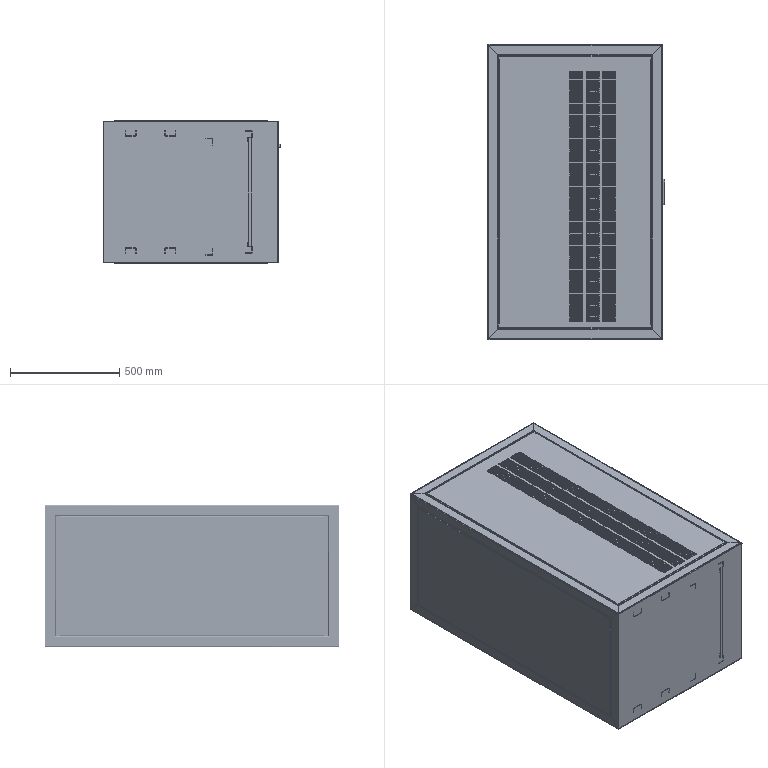Assembly | SolidWorks | mm | 39 component files | 39 solids | 4179 faces | box 814 x 1350 x 654 mm | volume 14968094 mm3 | plane 2169 | cylinder 1888 | spline 120 | torus 2 | commonest cylinder face diameters 5 x1380 8 x288 4 x90 6.4 x48 10 x28 6 x28 6.5 x12 7 x6
Bill of materials:
AuxiliaryPanel1 | 1 |  | Long thin-walled C-channel (lipped channel) profile with a flat web, two short flanges with rounded bends, and short inward-turned return lips; constant cross-section along its length.
AuxiliaryPanel2 | 1 |  | Long thin-walled lipped C-channel profile, similar to a sheet-formed channel, with flat web, rounded bends, short flanges and inward return lips; a single small round hole is visible near one end of a flange.
Beam1.1 | 1 |  | Straight angle profile (L-section) with two legs of roughly equal length joined by a rounded inside/outside bend; constant cross-section with plain square-cut ends.
Beam1.2 | 1 |  | Straight angle profile (L-section) with roughly equal legs and a radiused bend, shown with the corner facing the viewer; constant cross-section and plain ends.
Beam1.3 | 1 |  | Straight angle profile (L-section) with roughly equal legs and a radiused bend; plain ends, uniform cross-section.
Beam1.4 | 1 |  | Straight angle profile (L-section) with roughly equal legs and a radiused bend, corner facing the viewer; plain ends.
Beam1.5 | 1 |  | Straight angle profile (L-section) with roughly equal legs and a radiused bend, corner facing the viewer; plain ends.
Beam1.6 | 1 |  | Straight angle profile (L-section) with roughly equal legs and a radiused bend; plain ends, uniform cross-section.
BottomSupport | 3 |  | Long, thin rectangular flat bar or strip with small rounded or chamfered edges along its long sides; no holes or cut-outs visible.
FrontAndRearPlate1 | 1 |  | Thin sheet-formed Z-shaped (joggled) profile: two parallel offset flanges connected by a short web with rounded bends; the ends are cut at an angle so the outline narrows at the top and bottom.
FrontAndRearPlate2 | 1 |  | Thin sheet-formed Z-shaped (joggled) profile with angled cut ends, similar to unnamed part but mirrored in section; one small round hole near one end of a flange.
FrontAndRearPlate3 | 1 |  | Thin sheet-formed Z-shaped (joggled) profile with angled cut ends and one small round hole near one end of a flange; appears to be a mirrored or reoriented version of the other Z profiles.
FrontAndRearPlate4 | 1 |  | Elongated thin-walled strip with a joggled (Z-offset) cross-section: two parallel straight legs connected by a short perpendicular offset web with rounded bends; ends cut at an angle.
SupportChannelPlate | 4 |  | Long straight channel with a U-shaped (inverted U) open cross-section, rounded inside/outside corners, and square-cut ends.
SupportPlate1.1 | 1 |  | Long thin-walled profile with a multi-bend stepped cross-section (top lip, short horizontal return, tall web, bottom web, short upturned step, outward flange); ends mitered at an angle.
SupportPlate1.2 | 1 |  | Long thin-walled stepped multi-bend profile, apparently a mirrored or reoriented variant of the similar stepped section; ends mitered at an angle.
SupportPlate1.3 | 1 |  | Long thin-walled stepped multi-bend profile (outward flange, step up, top web, tall vertical web, inward return, downward lip) with ends mitered in the opposite sense, giving an inverted trapezoid in plan.
SupportPlate1 | 1 |  | Long thin-walled stepped multi-bend profile, mirror-like counterpart of the inverted-trapezoid variant, with angled (mitered) ends.
SupportPlate2.1 | 1 |  | Long straight thin-walled profile with an offset Z-like cross-section (vertical leg, horizontal offset, tall vertical web, horizontal bottom flange) with generous rounded bends and square-cut ends.
SupportPlate2.2 | 1 |  | Long straight thin-walled offset Z-like profile, apparently mirrored/rotated relative to the similar section, with rounded bends and square-cut ends.
SupportPlate3.1 | 1 |  | Long equal-or-near-equal leg angle (L-section) with a large inside bend radius and a single row of evenly spaced small round holes along one leg; square-cut ends.
SupportPlate3.2 | 1 |  | Long L-section angle with large rounded corner, a regular row of small holes along one leg, and a few additional sparse holes (single and paired) on the other leg; square-cut ends.
UpperAndLowerPlate(Lower) | 1 |  | Wide thin flat panel with a shallow C-shaped section: flat main web with short perpendicular flanges at both long edges, each ending in a small joggled/stepped return lip; ends mitered in plan.
UpperAndLowerPlate | 1 |  | Wide thin flat panel with short edge flanges at both long edges ending in small stepped/joggled lips facing the opposite side relative to the similar panel; ends mitered (trapezoidal in plan).
FanFixingPlate | 6 |  | Long, thin, flat rectangular bar with an elongated slot near each end and one round hole at the center.
FrontDoor | 1 |  | Thin rectangular plate with a small elongated raised boss or tab on one face near the middle of one long edge, and a small round feature at one edge corner in the side view.
LeftEndPlate | 1 |  | Large flat rectangular panel with three parallel columns of narrow slots (a vent pattern) set off-center, plus thin edge strips or lips along the long edges with small features at the corners.
RearDoor | 1 |  | Plain thin rectangular plate with narrow edge strips or lips along its two long edges and small notch-like features at the corners. It has no visible holes.
RightEndPlate | 1 |  | Large flat rectangular panel with three parallel columns of narrow slots (a vent pattern) set off-center, and small notch-like features at the corners of one edge.
Mates:
1. coincident | BoxWelding-1/SupportPlate3.2-1 face at (240.622, -44.499, 346.013) dir (0, 0, 1) | FanFixingPlate-1 face at (359.622, 55.501, 346.013) dir (0, 0, -1)
2. coincident | BoxWelding-1/SupportPlate3.2-1 axis at (254.622, 45.501, 344.013) dir (0, 0, 1) | FanFixingPlate-1 axis at (254.622, 45.501, 348.013) dir (0, 0, -1)
3. parallel | BoxWelding-1/UpperAndLowerPlate-1 face at (571.622, -44.499, -224.987) dir (0, 1, 0) | FanFixingPlate-1 face at (149.622, 35.501, 346.013) dir (0, -1, 0)
4. coincident | BoxWelding-1/SupportPlate3.2-1 face at (240.622, -44.499, 346.013) dir (0, 0, 1) | FanFixingPlate-2 face at (359.622, 243.501, 346.013) dir (0, 0, -1)
5. concentric | BoxWelding-1/SupportPlate3.2-1 face at (254.622, 233.501, 336.013) dir (0, 0, 1) r 3.2 | FanFixingPlate-2 face at (254.622, 233.501, 348.013) dir (0, 0, -1) r 3.25
6. concentric | BoxWelding-1/SupportPlate3.2-1 face at (254.622, 255.501, 336.013) dir (0, 0, 1) r 3.2 | FanFixingPlate-3 face at (254.622, 255.501, 348.013) dir (0, 0, -1) r 3.25
7. coincident | BoxWelding-1/SupportPlate3.2-1 face at (240.622, -44.499, 346.013) dir (0, 0, 1) | FanFixingPlate-3 face at (359.622, 265.501, 346.013) dir (0, 0, -1)
8. coincident | BoxWelding-1/SupportPlate3.2-1 face at (240.622, -44.499, 346.013) dir (0, 0, 1) | FanFixingPlate-4 face at (359.622, 455.501, 346.013) dir (0, 0, -1)
9. concentric | BoxWelding-1/SupportPlate3.2-1 face at (254.622, 445.501, 336.013) dir (0, 0, 1) r 3.2 | FanFixingPlate-4 face at (254.622, 445.501, 348.013) dir (0, 0, -1) r 3.25
10. coincident | BoxWelding-1/SupportPlate3.2-1 face at (240.622, -44.499, 346.013) dir (0, 0, 1) | FanFixingPlate-5 face at (359.622, 477.501, 346.013) dir (0, 0, -1)
11. concentric | BoxWelding-1/SupportPlate3.2-1 face at (254.622, 467.501, 336.013) dir (0, 0, 1) r 3.2 | FanFixingPlate-5 face at (254.622, 467.501, 348.013) dir (0, 0, -1) r 3.25
12. coincident | BoxWelding-1/SupportPlate3.2-1 face at (240.622, -44.499, 346.013) dir (0, 0, 1) | FanFixingPlate-6 face at (359.622, 667.501, 346.013) dir (0, 0, -1)
13. concentric | BoxWelding-1/SupportPlate3.2-1 face at (254.622, 657.501, 336.013) dir (0, 0, 1) r 3.2 | FanFixingPlate-6 face at (254.622, 657.501, 348.013) dir (0, 0, -1) r 3.25
14. parallel | BoxWelding-1/UpperAndLowerPlate-1 face at (571.622, -46.499, -224.987) dir (0, -1, 0) | FanFixingPlate-2 face at (149.622, 223.501, 346.013) dir (0, -1, 0)
15. parallel | BoxWelding-1/UpperAndLowerPlate-1 face at (571.622, -46.499, -224.987) dir (0, -1, 0) | FanFixingPlate-3 face at (149.622, 245.501, 346.013) dir (0, -1, 0)
16. parallel | BoxWelding-1/UpperAndLowerPlate-1 face at (571.622, -46.499, -224.987) dir (0, -1, 0) | FanFixingPlate-4 face at (149.622, 435.501, 346.013) dir (0, -1, 0)
17. parallel | BoxWelding-1/UpperAndLowerPlate-1 face at (571.622, -46.499, -224.987) dir (0, -1, 0) | FanFixingPlate-5 face at (149.622, 457.501, 346.013) dir (0, -1, 0)
18. parallel | BoxWelding-1/UpperAndLowerPlate-1 face at (571.622, -46.499, -224.987) dir (0, -1, 0) | FanFixingPlate-6 face at (149.622, 647.501, 346.013) dir (0, -1, 0)
19. concentric | BoxWelding-1/FrontAndRearPlate2-1 face at (561.622, -6.499, -164.987) dir (0, 1, 0) r 4 | FrontDoor-1 face at (561.622, 1253.506, -164.987) dir (0, -1, 0) r 4
20. coincident | BoxWelding-1/FrontAndRearPlate2-1 face at (569.622, 3.501, -224.987) dir (0, 1, 0) | FrontDoor-1 face at (571.622, 3.501, 372.513) dir (0, -1, 0)
21. coincident | BoxWelding-1/UpperAndLowerPlate-1 face at (571.622, 3.501, -206.987) dir (0, 0, -1) | LeftEndPlate-1 face at (521.622, 5.501, -206.987) dir (0, 0, 1)
22. coincident | BoxWelding-1/UpperAndLowerPlate-1 face at (-228.378, 3.501, -222.987) dir (0, 1, 0) | LeftEndPlate-1 face at (521.622, 3.501, -224.987) dir (0, -1, 0)
23. coincident | BoxWelding-1/SupportPlate1.2-1 face at (521.622, -44.499, -222.987) dir (-1, 0, 0) | LeftEndPlate-1 face at (521.622, 1233.501, -224.987) dir (1, 0, 0)
24. coincident | BoxWelding-1/UpperAndLowerPlate-1 face at (571.622, 3.501, 423.013) dir (0, 1, 0) | RightEndPlate-1 face at (-178.378, 3.501, 425.013) dir (0, -1, 0)
25. coincident | BoxWelding-1/SupportPlate1.3-1 face at (521.622, 1301.501, 423.013) dir (-1, 0, 0) | RightEndPlate-1 face at (521.622, 23.501, 425.013) dir (1, 0, 0)
26. coincident | BoxWelding-1/UpperAndLowerPlate-1 face at (-228.378, 3.501, 407.013) dir (0, 0, 1) | RightEndPlate-1 face at (-178.378, 5.501, 407.013) dir (0, 0, -1)
27. coincident | BoxWelding-1/FrontAndRearPlate1-1 face at (-226.378, 3.501, 425.013) dir (0, 1, 0) | RearDoor-2 face at (-228.378, 3.501, -174.987) dir (0, -1, 0)
28. coincident | BoxWelding-1/SupportPlate1-2 face at (-226.378, 1301.501, 375.013) dir (0, 0, -1) | RearDoor-2 face at (-228.378, 23.501, 375.013) dir (0, 0, 1)
29. coincident | BoxWelding-1/FrontAndRearPlate1-1 face at (-210.378, 3.501, -224.987) dir (-1, 0, 0) | RearDoor-2 face at (-210.378, 5.501, -174.987) dir (1, 0, 0)
30. coincident | BottomSupport-1 face at (579.856, 1348, -425.987) dir (1, 0, 0) | BottomSupport-2 face at (579.856, 1348, -685.987) dir (1, 0, 0)
31. distance | BottomSupport-2 face at (-140.144, 1348, -685.987) dir (0, 0, 1) | BottomSupport-1 face at (579.856, 1348, -525.987) dir (0, 0, -1)
32. coincident | BottomSupport-1 face at (579.856, 1348, -425.987) dir (1, 0, 0) | BottomSupport-3 face at (579.856, 1348, -165.987) dir (1, 0, 0)
33. distance | BottomSupport-3 face at (579.856, 1348, -265.987) dir (0, 0, -1) | BottomSupport-1 face at (-140.144, 1348, -425.987) dir (0, 0, 1)
34. coincident | UpperAndLowerPlate-1 face at (619.856, 2, -800.987) dir (0, 1, 0) | SupportPlate2.1-1 face at (482.856, 2, -720.987) dir (0, -1, 0)
35. coincident | UpperAndLowerPlate-1 face at (619.856, 2, -800.987) dir (0, 1, 0) | SupportPlate2.2-1 face at (494.856, 2, -200.987) dir (0, -1, 0)
36. coincident | SupportPlate2.1-1 face at (499.856, 2, -750.987) dir (1, 0, 0) | SupportPlate2.2-1 face at (499.856, 2, -200.987) dir (1, 0, 0)
37. distance | SupportPlate2.1-1 face at (468.856, 2, -755.987) dir (0, 0, -1) | BottomSupport-2 face at (579.856, 1348, -785.987) dir (0, 0, -1)
38. distance | SupportPlate2.2-1 face at (494.856, 2, -195.987) dir (0, 0, 1) | BottomSupport-3 face at (-140.144, 1348, -165.987) dir (0, 0, 1)
39. coincident | SupportPlate2.1-1 face at (479.856, 2, -720.987) dir (1, 0, 0) | AuxiliaryPanel1-1 face at (479.856, 4, -227.987) dir (-1, 0, 0)
40. coincident | UpperAndLowerPlate-1 face at (619.856, 2, -800.987) dir (0, 1, 0) | AuxiliaryPanel1-1 face at (497.856, 2, -227.987) dir (0, -1, 0)
41. coincident | SupportPlate2.1-1 face at (494.856, 2, -723.987) dir (0, 0, 1) | AuxiliaryPanel1-1 face at (497.856, 202, -723.987) dir (0, 0, -1)
42. coincident | SupportPlate2.1-1 face at (479.856, 2, -720.987) dir (1, 0, 0) | AuxiliaryPanel2-1 face at (479.856, 754, -227.987) dir (-1, 0, 0)
43. coincident | SupportPlate2.1-1 face at (494.856, 2, -723.987) dir (0, 0, 1) | AuxiliaryPanel2-1 face at (483.856, 756, -723.987) dir (0, 0, -1)
44. coincident | UpperAndLowerPlate-1 face at (619.856, 2, -800.987) dir (0, 1, 0) | SupportPlate3.1-1 face at (314.856, 2, -760.987) dir (0, -1, 0)
45. distance | SupportPlate3.1-1 face at (288.856, 2, -765.987) dir (0, 0, -1) | BottomSupport-2 face at (579.856, 1348, -785.987) dir (0, 0, -1)
46. coincident | UpperAndLowerPlate-1 face at (619.856, 2, -800.987) dir (0, 1, 0) | SupportPlate3.2-1 face at (314.856, 2, -234.987) dir (0, -1, 0)
47. coincident | SupportPlate3.1-1 face at (319.856, 2, -760.987) dir (1, 0, 0) | SupportPlate3.2-1 face at (319.856, 2, -234.987) dir (1, 0, 0)
48. distance | SupportPlate3.2-1 face at (288.856, 2, -229.987) dir (0, 0, 1) | BottomSupport-3 face at (-140.144, 1348, -165.987) dir (0, 0, 1)
49. coincident | UpperAndLowerPlate-1 face at (619.856, 2, -800.987) dir (0, 1, 0) | SupportChannelPlate-1 face at (-35.144, 2, -735.987) dir (0, -1, 0)
50. distance | SupportChannelPlate-1 face at (-30.144, 2, -755.987) dir (0, 0, -1) | BottomSupport-2 face at (579.856, 1348, -785.987) dir (0, 0, -1)
51. coincident | SupportChannelPlate-1 face at (-35.144, 2, -730.987) dir (0, 0, 1) | SupportChannelPlate-2 face at (144.856, 2, -730.987) dir (0, 0, 1)
52. coincident | UpperAndLowerPlate-1 face at (619.856, 2, -800.987) dir (0, 1, 0) | SupportChannelPlate-2 face at (144.856, 2, -735.987) dir (0, -1, 0)
53. distance | SupportChannelPlate-2 face at (99.856, 2, -755.987) dir (-1, 0, 0) | SupportChannelPlate-1 face at (-30.144, 2, -755.987) dir (1, 0, 0)
54. coincident | UpperAndLowerPlate-1 face at (619.856, 2, -800.987) dir (0, 1, 0) | SupportChannelPlate-3 face at (104.856, 2, -215.987) dir (0, -1, 0)
55. distance | SupportChannelPlate-3 face at (99.856, 2, -195.987) dir (0, 0, 1) | BottomSupport-3 face at (-140.144, 1348, -165.987) dir (0, 0, 1)
56. coincident | UpperAndLowerPlate-1 face at (619.856, 2, -800.987) dir (0, 1, 0) | SupportChannelPlate-4 face at (-75.144, 2, -215.987) dir (0, -1, 0)
57. coincident | UpperAndLowerPlate-1 face at (619.856, 2, -800.987) dir (0, 1, 0) | SupportChannelPlate-4 face at (-75.144, 2, -215.987) dir (0, -1, 0)
58. coincident | SupportChannelPlate-1 face at (-80.144, 2, -755.987) dir (-1, 0, 0) | SupportChannelPlate-4 face at (-80.144, 2, -195.987) dir (-1, 0, 0)
59. distance | SupportChannelPlate-4 face at (-32.144, 2, -195.987) dir (0, 0, 1) | BottomSupport-3 face at (-140.144, 1348, -165.987) dir (0, 0, 1)
60. distance | SupportChannelPlate-4 face at (-30.144, 2, -195.987) dir (1, 0, 0) | SupportChannelPlate-3 face at (99.856, 2, -195.987) dir (-1, 0, 0)
61. coincident | SupportChannelPlate-3 face at (104.856, 2, -220.987) dir (0, 0, -1) | Beam1.1-1 face at (111.356, 839.5, -220.987) dir (0, 0, 1)
62. distance | Beam1.1-1 face at (104.856, 873, -220.987) dir (-1, 0, 0) | SupportChannelPlate-3 face at (99.856, 2, -195.987) dir (-1, 0, 0)
63. coincident | Beam1.1-1 face at (111.356, 833, -220.987) dir (0, -1, 0) | Beam1.2-1 face at (-41.644, 833, -730.987) dir (0, -1, 0)
64. coincident | SupportChannelPlate-4 face at (-75.144, 2, -220.987) dir (0, 0, -1) | Beam1.2-1 face at (-41.644, 839.5, -220.987) dir (0, 0, 1)
65. distance | Beam1.2-1 face at (-75.144, 836, -730.987) dir (-1, 0, 0) | SupportChannelPlate-4 face at (-80.144, 2, -195.987) dir (-1, 0, 0)
66. coincident | SupportChannelPlate-3 face at (104.856, 2, -220.987) dir (0, 0, -1) | Beam1.3-1 face at (111.356, 574.5, -220.987) dir (0, 0, 1)
67. distance | Beam1.3-1 face at (104.856, 608, -220.987) dir (-1, 0, 0) | SupportChannelPlate-3 face at (99.856, 2, -195.987) dir (-1, 0, 0)
68. distance | Beam1.3-1 face at (111.356, 568, -220.987) dir (0, -1, 0) | Beam1.1-1 face at (111.356, 833, -220.987) dir (0, -1, 0)
69. coincident | Beam1.3-1 face at (111.356, 568, -220.987) dir (0, -1, 0) | Beam1.4-1 face at (-75.144, 568, -220.987) dir (0, -1, 0)
70. coincident | SupportChannelPlate-4 face at (-75.144, 2, -220.987) dir (0, 0, -1) | Beam1.4-1 face at (-41.644, 574.5, -220.987) dir (0, 0, 1)
71. distance | Beam1.4-1 face at (-75.144, 568, -220.987) dir (-1, 0, 0) | SupportChannelPlate-4 face at (-80.144, 2, -195.987) dir (-1, 0, 0)
72. distance | BottomSupport-2 face at (579.856, 1348, -685.987) dir (1, 0, 0) | FrontAndRearPlate3-1 face at (619.856, 1300, -800.987) dir (1, 0, 0)
73. coincident | BottomSupport-3 face at (579.856, 1348, -265.987) dir (0, 1, 0) | UpperAndLowerPlate(Lower)-1 face at (619.856, 1348, -150.987) dir (0, -1, 0)
74. coincident | BottomSupport-2 face at (-140.144, 1348, -685.987) dir (0, 1, 0) | UpperAndLowerPlate(Lower)-1 face at (619.856, 1348, -150.987) dir (0, -1, 0)
75. coincident | BottomSupport-1 face at (579.856, 1348, -525.987) dir (0, 1, 0) | UpperAndLowerPlate(Lower)-1 face at (619.856, 1348, -150.987) dir (0, -1, 0)
76. coincident | BottomSupport-1 plane at (219.856, 1334.5, -475.987) dir (0, 0, 1) | UpperAndLowerPlate(Lower)-1 plane at (219.856, 1349, -475.987) dir (0, 0, -1)
77. distance | SupportPlate2.1-1 face at (499.856, 2, -750.987) dir (1, 0, 0) | FrontAndRearPlate3-1 face at (619.856, 1300, -800.987) dir (1, 0, 0)
78. distance | SupportPlate3.2-1 face at (319.856, 2, -234.987) dir (1, 0, 0) | FrontAndRearPlate3-1 face at (619.856, 1300, -800.987) dir (1, 0, 0)
79. distance | Beam1.2-1 face at (-41.644, 833, -730.987) dir (0, -1, 0) | BottomSupport-1 face at (579.856, 1333, -425.987) dir (0, -1, 0)
80. coincident | UpperAndLowerPlate-1 face at (-180.144, 2, -800.987) dir (0, 0, -1) | SupportPlate1.1-1 face at (-180.144, 2, -800.987) dir (0, 0, -1)
81. coincident | UpperAndLowerPlate-1 face at (-180.144, 0, -800.987) dir (-0.7071, 0.7071, 0) | SupportPlate1.1-1 face at (-178.144, 2, -800.987) dir (0.7071, -0.7071, 0)
82. coincident | UpperAndLowerPlate-1 edge at (-112.144, 68, -782.987) dir (0, 0, 1) | SupportPlate1.1-1 edge at (-112.144, 68, -780.987) dir (0, 0, -1)
83. coincident | UpperAndLowerPlate-1 face at (-180.144, 2, -800.987) dir (0, 0, -1) | SupportPlate1.2-1 face at (617.856, 2, -800.987) dir (0, 0, -1)
84. coincident | UpperAndLowerPlate(Lower)-1 face at (619.856, 1348, -800.987) dir (0, 0, -1) | SupportPlate1.1-1 face at (-180.144, 2, -800.987) dir (0, 0, -1)
85. coincident | UpperAndLowerPlate(Lower)-1 face at (220.856, 949, -798.987) dir (-0.7071, -0.7071, 0) | SupportPlate1.1-1 face at (493.856, 676, -798.987) dir (0.7071, 0.7071, 0)
86. coincident | UpperAndLowerPlate(Lower)-1 edge at (-112.144, 1282, -780.987) dir (0, 0, -1) | SupportPlate1.1-1 edge at (-112.144, 1282, -782.987) dir (0, 0, 1)
87. coincident | UpperAndLowerPlate-1 face at (-180.144, 2, -800.987) dir (0, 0, -1) | SupportPlate1.2-1 face at (617.856, 2, -800.987) dir (0, 0, -1)
88. coincident | FrontAndRearPlate2-1 face at (619.856, 50, -150.987) dir (1, 0, 0) | SupportPlate1.2-1 face at (619.856, 2, -800.987) dir (1, 0, 0)
89. coincident | UpperAndLowerPlate-1 face at (218.856, 401, -798.987) dir (0.7071, 0.7071, 0) | SupportPlate1.2-1 face at (617.856, 2, -800.987) dir (-0.7071, -0.7071, 0)
90. coincident | UpperAndLowerPlate-1 edge at (551.856, 68, -780.987) dir (0, 0, -1) | SupportPlate1.2-1 edge at (551.856, 68, -782.987) dir (0, 0, 1)
91. coincident | FrontAndRearPlate2-1 face at (619.856, 50, -150.987) dir (1, 0, 0) | SupportPlate1.2-1 face at (619.856, 2, -800.987) dir (1, 0, 0)
92. coincident | FrontAndRearPlate2-1 face at (601.856, 350, -450.987) dir (0, 0.7071, -0.7071) | SupportPlate1.2-1 face at (599.856, 2, -798.987) dir (0, -0.7071, 0.7071)
93. coincident | FrontAndRearPlate2-1 edge at (601.856, 68, -732.987) dir (-1, 0, 0) | SupportPlate1.2-1 edge at (599.856, 68, -732.987) dir (1, 0, 0)
94. coincident | FrontAndRearPlate2-1 face at (619.856, 50, -150.987) dir (1, 0, 0) | SupportPlate1.3-1 face at (619.856, 1348, -150.987) dir (1, 0, 0)
95. coincident | UpperAndLowerPlate-1 face at (619.856, 2, -150.987) dir (0, 0, 1) | SupportPlate1.3-1 face at (617.856, 1348, -150.987) dir (0, 0, 1)
96. coincident | UpperAndLowerPlate-1 face at (619.856, 0, -150.987) dir (0.7071, 0.7071, 0) | SupportPlate1.3-1 face at (-55.144, 675, -152.987) dir (-0.7071, -0.7071, 0)
97. coincident | FrontAndRearPlate3-1 face at (619.856, 1300, -800.987) dir (1, 0, 0) | SupportPlate1.2-1 face at (619.856, 2, -800.987) dir (1, 0, 0)
98. coincident | UpperAndLowerPlate-1 face at (619.856, 2, -150.987) dir (0, 0, 1) | SupportPlate1-2 face at (-178.144, 2, -150.987) dir (0, 0, 1)
99. coincident | SupportPlate1-2 face at (-180.144, 2, -150.987) dir (-1, 0, 0) | FrontAndRearPlate1-1 face at (-180.144, 50, -800.987) dir (-1, 0, 0)
100. coincident | UpperAndLowerPlate-1 face at (220.856, 401, -152.987) dir (-0.7071, 0.7071, 0) | SupportPlate1-2 face at (-178.144, 2, -150.987) dir (0.7071, -0.7071, 0)
101. coincident | UpperAndLowerPlate-1 edge at (-112.144, 68, -169.987) dir (1, 0, 0) | SupportPlate1-2 edge at (-112.144, 68, -168.987) dir (0, 0, -1)
102. coincident | SupportPlate1-2 face at (-180.144, 2, -150.987) dir (-1, 0, 0) | FrontAndRearPlate1-1 face at (-180.144, 50, -800.987) dir (-1, 0, 0)
103. coincident | SupportPlate1-2 face at (-180.144, 2, -152.987) dir (0, -0.7071, -0.7071) | FrontAndRearPlate1-1 face at (-178.144, 350, -500.987) dir (0, 0.7071, 0.7071)
104. coincident | SupportPlate1-2 edge at (-160.144, 68, -218.987) dir (-1, 0, 0) | FrontAndRearPlate1-1 edge at (-162.144, 68, -218.987) dir (1, 0, 0)
105. coincident | SupportPlate1-2 face at (-180.144, 2, -150.987) dir (-1, 0, 0) | FrontAndRearPlate4-1 face at (-180.144, 1300, -150.987) dir (-1, 0, 0)
106. coincident | SupportPlate1-2 face at (-178.144, 676, -824.987) dir (0, 0.7071, -0.7071) | FrontAndRearPlate4-1 face at (-178.144, 1325, -175.987) dir (0, -0.7071, 0.7071)
107. coincident | SupportPlate1-2 face at (-160.144, 2, -218.987) dir (0, 0, -1) | FrontAndRearPlate4-1 edge at (-160.144, 1282, -218.987) dir (-1, 0, 0)
108. distance | SupportChannelPlate-1 face at (-80.144, 2, -755.987) dir (-1, 0, 0) | FrontAndRearPlate4-1 face at (-180.144, 1300, -150.987) dir (-1, 0, 0)
109. distance | AuxiliaryPanel2-1 face at (497.856, 752, -227.987) dir (0, -1, 0) | AuxiliaryPanel1-1 face at (497.856, 202, -723.987) dir (0, 1, 0)
110. coincident | SupportChannelPlate-3 face at (104.856, 2, -220.987) dir (0, 0, -1) | Beam1.6-1 face at (111.356, 309.5, -220.987) dir (0, 0, 1)
111. coincident | Beam1.3-1 face at (104.856, 608, -220.987) dir (-1, 0, 0) | Beam1.6-1 face at (104.856, 343, -220.987) dir (-1, 0, 0)
112. distance | Beam1.6-1 face at (111.356, 303, -220.987) dir (0, -1, 0) | Beam1.3-1 face at (111.356, 568, -220.987) dir (0, -1, 0)
113. coincident | Beam1.5-1 face at (-41.644, 303, -730.987) dir (0, -1, 0) | Beam1.6-1 face at (111.356, 303, -220.987) dir (0, -1, 0)
114. coincident | SupportChannelPlate-4 face at (-75.144, 2, -220.987) dir (0, 0, -1) | Beam1.5-1 face at (-41.644, 309.5, -220.987) dir (0, 0, 1)
115. coincident | Beam1.4-1 face at (-35.144, 574.5, -220.987) dir (1, 0, 0) | Beam1.5-1 face at (-35.144, 343, -730.987) dir (1, 0, 0)
116. coincident | FrontAndRearPlate3-1 edge at (599.856, 1282, -732.987) dir (1, 0, 0) | SupportPlate1.2-1 edge at (601.856, 1282, -732.987) dir (-1, 0, 0)
117. coincident | UpperAndLowerPlate-1 face at (619.856, 0, -800.987) dir (0, -1, 0) | BoxWelding plane at (0, 0, 0) dir (0, 1, 0)